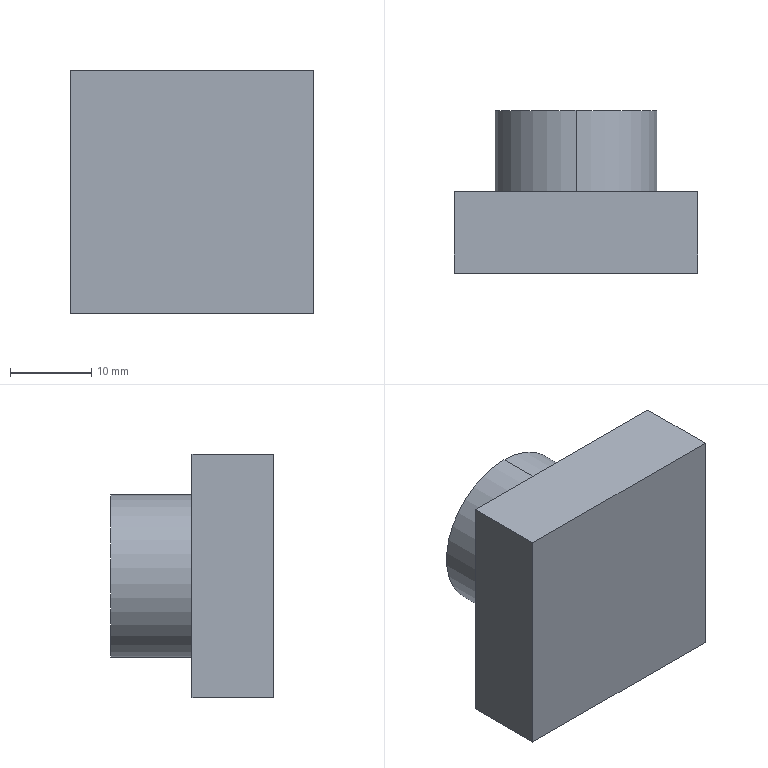Component | SolidWorks | Workpiece-2 | 1 solid | 9 faces | box 30 x 20 x 30 mm | volume 12142 mm3 | plane 7 | cylinder 2 | commonest cylinder face diameters 20 x2
build123d program:
from build123d import *

# Parameters (mm, degrees)
SKETCH2_W           = 30
SKETCH2_H           = 30
BOSS_EXTRUDE1_DEPTH = 10
SKETCH3_R           = 10
BOSS_EXTRUDE2_DEPTH = 10


with BuildPart() as part:
    # Sketch2 → Boss-Extrude1 (new body)
    with BuildSketch(Plane.XY):
        with Locations((-70.975, 8.462)):
            Rectangle(SKETCH2_W, SKETCH2_H)
    extrude(amount=BOSS_EXTRUDE1_DEPTH)

    # Sketch3 → Boss-Extrude2 (add)
    with BuildSketch(Plane.XY.offset(10)):
        with Locations((-70.975, 8.462)):
            Circle(SKETCH3_R)
    extrude(amount=BOSS_EXTRUDE2_DEPTH)


solid = part.part

# Placed as in the assembly
solid = solid.moved(Location((-78.951, 112, 8.462), (-90, 0, 0)))
STEP:
#1=COLOUR_RGB('',0.7922,0.8196,0.9333);
#2=FILL_AREA_STYLE_COLOUR('',#1);
#3=FILL_AREA_STYLE('',(#2));
#4=SURFACE_STYLE_FILL_AREA(#3);
#5=SURFACE_SIDE_STYLE('',(#4));
#6=SURFACE_STYLE_USAGE(.BOTH.,#5);
#7=PRESENTATION_STYLE_ASSIGNMENT((#6));
#8=CARTESIAN_POINT('',(-5.903,5.197,-0.3937));
#9=VERTEX_POINT('',#8);
#10=CARTESIAN_POINT('',(-5.903,5.197,0.3937));
#11=VERTEX_POINT('',#10);
#12=CARTESIAN_POINT('',(-5.903,5.197,0.));
#13=DIRECTION('',(0.,1.,0.));
#14=DIRECTION('',(0.,0.,-1.));
#15=AXIS2_PLACEMENT_3D('',#12,#13,#14);
#16=CIRCLE('',#15,0.3937);
#17=EDGE_CURVE('',#9,#11,#16,.T.);
#18=ORIENTED_EDGE('',*,*,#17,.F.);
#19=CARTESIAN_POINT('',(-5.903,4.803,-0.3937));
#20=VERTEX_POINT('',#19);
#21=CARTESIAN_POINT('',(-5.903,5.197,-0.3937));
#22=DIRECTION('',(-0.,-1.,0.));
#23=VECTOR('',#22,39.37);
#24=LINE('',#21,#23);
#25=EDGE_CURVE('',#9,#20,#24,.T.);
#26=ORIENTED_EDGE('',*,*,#25,.T.);
#27=CARTESIAN_POINT('',(-5.903,4.803,0.3937));
#28=VERTEX_POINT('',#27);
#29=CARTESIAN_POINT('',(-5.903,4.803,0.));
#30=DIRECTION('',(0.,1.,0.));
#31=DIRECTION('',(0.,0.,-1.));
#32=AXIS2_PLACEMENT_3D('',#29,#30,#31);
#33=CIRCLE('',#32,0.3937);
#34=EDGE_CURVE('',#20,#28,#33,.T.);
#35=ORIENTED_EDGE('',*,*,#34,.T.);
#36=CARTESIAN_POINT('',(-5.903,5.197,0.3937));
#37=DIRECTION('',(-0.,-1.,0.));
#38=VECTOR('',#37,39.37);
#39=LINE('',#36,#38);
#40=EDGE_CURVE('',#11,#28,#39,.T.);
#41=ORIENTED_EDGE('',*,*,#40,.F.);
#42=EDGE_LOOP('',(#18,#26,#35,#41));
#43=FACE_OUTER_BOUND('',#42,.T.);
#44=CARTESIAN_POINT('',(-5.903,5.197,0.));
#45=DIRECTION('',(-0.,-1.,0.));
#46=DIRECTION('',(0.,0.,1.));
#47=AXIS2_PLACEMENT_3D('',#44,#45,#46);
#48=CYLINDRICAL_SURFACE('',#47,0.3937);
#49=ADVANCED_FACE('',(#43),#48,.T.);
#50=CARTESIAN_POINT('',(-5.312,4.409,-0.5906));
#51=VERTEX_POINT('',#50);
#52=CARTESIAN_POINT('',(-6.493,4.409,-0.5906));
#53=VERTEX_POINT('',#52);
#54=CARTESIAN_POINT('',(-6.493,4.409,-0.5906));
#55=DIRECTION('',(-1.,0.,0.));
#56=VECTOR('',#55,39.37);
#57=LINE('',#54,#56);
#58=EDGE_CURVE('',#51,#53,#57,.T.);
#59=ORIENTED_EDGE('',*,*,#58,.T.);
#60=CARTESIAN_POINT('',(-6.493,4.803,-0.5906));
#61=VERTEX_POINT('',#60);
#62=CARTESIAN_POINT('',(-6.493,4.803,-0.5906));
#63=DIRECTION('',(-0.,-1.,0.));
#64=VECTOR('',#63,39.37);
#65=LINE('',#62,#64);
#66=EDGE_CURVE('',#61,#53,#65,.T.);
#67=ORIENTED_EDGE('',*,*,#66,.F.);
#68=CARTESIAN_POINT('',(-5.312,4.803,-0.5906));
#69=VERTEX_POINT('',#68);
#70=CARTESIAN_POINT('',(-6.493,4.803,-0.5906));
#71=DIRECTION('',(-1.,0.,0.));
#72=VECTOR('',#71,39.37);
#73=LINE('',#70,#72);
#74=EDGE_CURVE('',#69,#61,#73,.T.);
#75=ORIENTED_EDGE('',*,*,#74,.F.);
#76=CARTESIAN_POINT('',(-5.312,4.803,-0.5906));
#77=DIRECTION('',(-0.,-1.,0.));
#78=VECTOR('',#77,39.37);
#79=LINE('',#76,#78);
#80=EDGE_CURVE('',#69,#51,#79,.T.);
#81=ORIENTED_EDGE('',*,*,#80,.T.);
#82=EDGE_LOOP('',(#59,#67,#75,#81));
#83=FACE_OUTER_BOUND('',#82,.T.);
#84=CARTESIAN_POINT('',(-6.493,4.803,-0.5906));
#85=DIRECTION('',(0.,0.,1.));
#86=DIRECTION('',(0.,1.,0.));
#87=AXIS2_PLACEMENT_3D('',#84,#85,#86);
#88=PLANE('',#87);
#89=ADVANCED_FACE('',(#83),#88,.F.);
#90=CARTESIAN_POINT('',(-6.493,4.409,0.5906));
#91=VERTEX_POINT('',#90);
#92=CARTESIAN_POINT('',(-6.493,4.409,-0.5906));
#93=DIRECTION('',(0.,-0.,1.));
#94=VECTOR('',#93,39.37);
#95=LINE('',#92,#94);
#96=EDGE_CURVE('',#53,#91,#95,.T.);
#97=ORIENTED_EDGE('',*,*,#96,.T.);
#98=CARTESIAN_POINT('',(-6.493,4.803,0.5906));
#99=VERTEX_POINT('',#98);
#100=CARTESIAN_POINT('',(-6.493,4.803,0.5906));
#101=DIRECTION('',(-0.,-1.,0.));
#102=VECTOR('',#101,39.37);
#103=LINE('',#100,#102);
#104=EDGE_CURVE('',#99,#91,#103,.T.);
#105=ORIENTED_EDGE('',*,*,#104,.F.);
#106=CARTESIAN_POINT('',(-6.493,4.803,-0.5906));
#107=DIRECTION('',(0.,-0.,1.));
#108=VECTOR('',#107,39.37);
#109=LINE('',#106,#108);
#110=EDGE_CURVE('',#61,#99,#109,.T.);
#111=ORIENTED_EDGE('',*,*,#110,.F.);
#112=ORIENTED_EDGE('',*,*,#66,.T.);
#113=EDGE_LOOP('',(#97,#105,#111,#112));
#114=FACE_OUTER_BOUND('',#113,.T.);
#115=CARTESIAN_POINT('',(-6.493,4.803,-0.5906));
#116=DIRECTION('',(1.,-0.,-0.));
#117=DIRECTION('',(-0.,0.,-1.));
#118=AXIS2_PLACEMENT_3D('',#115,#116,#117);
#119=PLANE('',#118);
#120=ADVANCED_FACE('',(#114),#119,.F.);
#121=CARTESIAN_POINT('',(-5.312,4.409,0.5906));
#122=VERTEX_POINT('',#121);
#123=CARTESIAN_POINT('',(-6.493,4.409,0.5906));
#124=DIRECTION('',(1.,-0.,0.));
#125=VECTOR('',#124,39.37);
#126=LINE('',#123,#125);
#127=EDGE_CURVE('',#91,#122,#126,.T.);
#128=ORIENTED_EDGE('',*,*,#127,.T.);
#129=CARTESIAN_POINT('',(-5.312,4.803,0.5906));
#130=VERTEX_POINT('',#129);
#131=CARTESIAN_POINT('',(-5.312,4.803,0.5906));
#132=DIRECTION('',(-0.,-1.,0.));
#133=VECTOR('',#132,39.37);
#134=LINE('',#131,#133);
#135=EDGE_CURVE('',#130,#122,#134,.T.);
#136=ORIENTED_EDGE('',*,*,#135,.F.);
#137=CARTESIAN_POINT('',(-6.493,4.803,0.5906));
#138=DIRECTION('',(1.,-0.,0.));
#139=VECTOR('',#138,39.37);
#140=LINE('',#137,#139);
#141=EDGE_CURVE('',#99,#130,#140,.T.);
#142=ORIENTED_EDGE('',*,*,#141,.F.);
#143=ORIENTED_EDGE('',*,*,#104,.T.);
#144=EDGE_LOOP('',(#128,#136,#142,#143));
#145=FACE_OUTER_BOUND('',#144,.T.);
#146=CARTESIAN_POINT('',(-6.493,4.803,0.5906));
#147=DIRECTION('',(0.,0.,-1.));
#148=DIRECTION('',(-0.,-1.,0.));
#149=AXIS2_PLACEMENT_3D('',#146,#147,#148);
#150=PLANE('',#149);
#151=ADVANCED_FACE('',(#145),#150,.F.);
#152=CARTESIAN_POINT('',(-5.312,4.409,-0.5906));
#153=DIRECTION('',(0.,0.,-1.));
#154=VECTOR('',#153,39.37);
#155=LINE('',#152,#154);
#156=EDGE_CURVE('',#122,#51,#155,.T.);
#157=ORIENTED_EDGE('',*,*,#156,.T.);
#158=ORIENTED_EDGE('',*,*,#80,.F.);
#159=CARTESIAN_POINT('',(-5.312,4.803,-0.5906));
#160=DIRECTION('',(0.,0.,-1.));
#161=VECTOR('',#160,39.37);
#162=LINE('',#159,#161);
#163=EDGE_CURVE('',#130,#69,#162,.T.);
#164=ORIENTED_EDGE('',*,*,#163,.F.);
#165=ORIENTED_EDGE('',*,*,#135,.T.);
#166=EDGE_LOOP('',(#157,#158,#164,#165));
#167=FACE_OUTER_BOUND('',#166,.T.);
#168=CARTESIAN_POINT('',(-5.312,4.803,-0.5906));
#169=DIRECTION('',(-1.,0.,0.));
#170=DIRECTION('',(0.,1.,0.));
#171=AXIS2_PLACEMENT_3D('',#168,#169,#170);
#172=PLANE('',#171);
#173=ADVANCED_FACE('',(#167),#172,.F.);
#174=CARTESIAN_POINT('',(-5.903,4.803,0.));
#175=DIRECTION('',(0.,1.,0.));
#176=DIRECTION('',(0.,0.,-1.));
#177=AXIS2_PLACEMENT_3D('',#174,#175,#176);
#178=CIRCLE('',#177,0.3937);
#179=EDGE_CURVE('',#28,#20,#178,.T.);
#180=ORIENTED_EDGE('',*,*,#179,.F.);
#181=ORIENTED_EDGE('',*,*,#34,.F.);
#182=EDGE_LOOP('',(#180,#181));
#183=FACE_BOUND('',#182,.T.);
#184=ORIENTED_EDGE('',*,*,#74,.T.);
#185=ORIENTED_EDGE('',*,*,#110,.T.);
#186=ORIENTED_EDGE('',*,*,#141,.T.);
#187=ORIENTED_EDGE('',*,*,#163,.T.);
#188=EDGE_LOOP('',(#184,#185,#186,#187));
#189=FACE_OUTER_BOUND('',#188,.T.);
#190=CARTESIAN_POINT('',(-5.569,4.803,-2.794));
#191=DIRECTION('',(-0.,-1.,0.));
#192=DIRECTION('',(0.,0.,1.));
#193=AXIS2_PLACEMENT_3D('',#190,#191,#192);
#194=PLANE('',#193);
#195=ADVANCED_FACE('',(#183,#189),#194,.F.);
#196=ORIENTED_EDGE('',*,*,#58,.F.);
#197=ORIENTED_EDGE('',*,*,#156,.F.);
#198=ORIENTED_EDGE('',*,*,#127,.F.);
#199=ORIENTED_EDGE('',*,*,#96,.F.);
#200=EDGE_LOOP('',(#196,#197,#198,#199));
#201=FACE_OUTER_BOUND('',#200,.T.);
#202=CARTESIAN_POINT('',(-5.569,4.409,-2.794));
#203=DIRECTION('',(-0.,-1.,0.));
#204=DIRECTION('',(0.,0.,1.));
#205=AXIS2_PLACEMENT_3D('',#202,#203,#204);
#206=PLANE('',#205);
#207=ADVANCED_FACE('',(#201),#206,.T.);
#208=ORIENTED_EDGE('',*,*,#25,.F.);
#209=CARTESIAN_POINT('',(-5.903,5.197,0.));
#210=DIRECTION('',(0.,1.,0.));
#211=DIRECTION('',(0.,0.,-1.));
#212=AXIS2_PLACEMENT_3D('',#209,#210,#211);
#213=CIRCLE('',#212,0.3937);
#214=EDGE_CURVE('',#11,#9,#213,.T.);
#215=ORIENTED_EDGE('',*,*,#214,.F.);
#216=ORIENTED_EDGE('',*,*,#40,.T.);
#217=ORIENTED_EDGE('',*,*,#179,.T.);
#218=EDGE_LOOP('',(#208,#215,#216,#217));
#219=FACE_OUTER_BOUND('',#218,.T.);
#220=CARTESIAN_POINT('',(-5.903,5.197,0.));
#221=DIRECTION('',(-0.,-1.,0.));
#222=DIRECTION('',(0.,0.,1.));
#223=AXIS2_PLACEMENT_3D('',#220,#221,#222);
#224=CYLINDRICAL_SURFACE('',#223,0.3937);
#225=ADVANCED_FACE('',(#219),#224,.T.);
#226=ORIENTED_EDGE('',*,*,#214,.T.);
#227=ORIENTED_EDGE('',*,*,#17,.T.);
#228=EDGE_LOOP('',(#226,#227));
#229=FACE_OUTER_BOUND('',#228,.T.);
#230=CARTESIAN_POINT('',(-5.903,5.197,0.));
#231=DIRECTION('',(0.,1.,0.));
#232=DIRECTION('',(0.,0.,-1.));
#233=AXIS2_PLACEMENT_3D('',#230,#231,#232);
#234=PLANE('',#233);
#235=ADVANCED_FACE('',(#229),#234,.T.);
#236=CLOSED_SHELL('',(#49,#89,#120,#151,#173,#195,#207,#225,#235));
#237=MANIFOLD_SOLID_BREP('',#236);
#238=STYLED_ITEM('',(#7),#237);
#239=PRESENTATION_LAYER_ASSIGNMENT('','',(#238));
#240=CARTESIAN_POINT('',(0.,0.,0.));
#241=DIRECTION('',(0.,0.,1.));
#242=DIRECTION('',(1.,0.,0.));
#243=AXIS2_PLACEMENT_3D('',#240,#241,#242);
#244=(LENGTH_UNIT()NAMED_UNIT(*)SI_UNIT($,.METRE.));
#245=LENGTH_MEASURE_WITH_UNIT(LENGTH_MEASURE(0.0254),#244);
#246=DIMENSIONAL_EXPONENTS(1.,0.,0.,0.,0.,0.,0.);
#247=(CONVERSION_BASED_UNIT('',#245)LENGTH_UNIT()NAMED_UNIT(#246));
#248=UNCERTAINTY_MEASURE_WITH_UNIT(LENGTH_MEASURE(0.00001),#247,'','');
#249=(NAMED_UNIT(*)PLANE_ANGLE_UNIT()SI_UNIT($,.RADIAN.));
#250=(NAMED_UNIT(*)SI_UNIT($,.STERADIAN.)SOLID_ANGLE_UNIT());
#251=(GEOMETRIC_REPRESENTATION_CONTEXT(3)GLOBAL_UNCERTAINTY_ASSIGNED_CONTEXT((#248))GLOBAL_UNIT_ASSIGNED_CONTEXT((#247,#249,#250))REPRESENTATION_CONTEXT('',''));
#252=ADVANCED_BREP_SHAPE_REPRESENTATION('',(#237,#243),#251);
#253=(LENGTH_UNIT()NAMED_UNIT(*)SI_UNIT($,.METRE.));
#254=LENGTH_MEASURE_WITH_UNIT(LENGTH_MEASURE(0.0254),#253);
#255=DIMENSIONAL_EXPONENTS(1.,0.,0.,0.,0.,0.,0.);
#256=(CONVERSION_BASED_UNIT('',#254)LENGTH_UNIT()NAMED_UNIT(#255));
#257=UNCERTAINTY_MEASURE_WITH_UNIT(LENGTH_MEASURE(0.00001),#256,'','');
#258=(NAMED_UNIT(*)PLANE_ANGLE_UNIT()SI_UNIT($,.RADIAN.));
#259=(NAMED_UNIT(*)SI_UNIT($,.STERADIAN.)SOLID_ANGLE_UNIT());
#260=(GEOMETRIC_REPRESENTATION_CONTEXT(3)GLOBAL_UNCERTAINTY_ASSIGNED_CONTEXT((#257))GLOBAL_UNIT_ASSIGNED_CONTEXT((#256,#258,#259))REPRESENTATION_CONTEXT('',''));
#261=MECHANICAL_DESIGN_GEOMETRIC_PRESENTATION_REPRESENTATION('',(#238),#260);